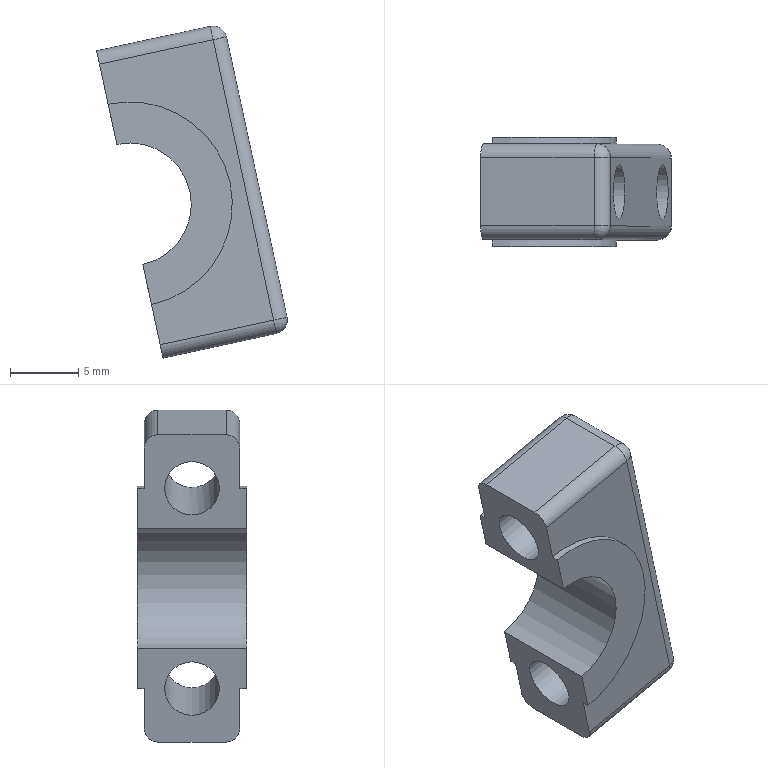Component | NX | CONNECTING_ROD_1_LOWER_BLOCK_2 | 1 solid | 26 faces | volume 1104 mm3 | cylinder 13 | plane 9 | sphere 4 | commonest cylinder face diameters 2 x8 15 x2 4 x2 9 x1